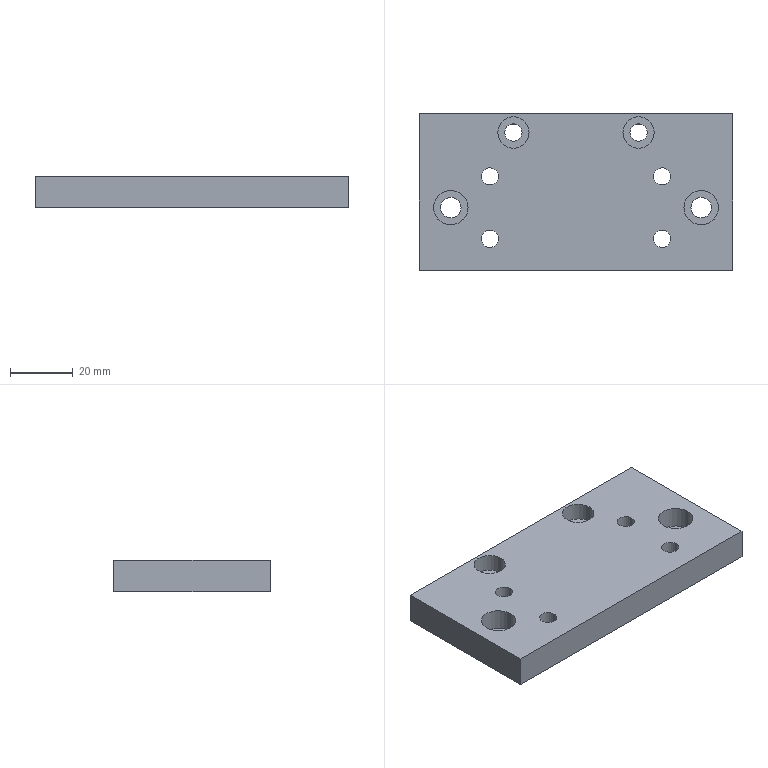Component | SolidWorks | 75-02-18StirringMotorMountingPlateModified-1 | 1 solid | 46 faces | box 100 x 50 x 10 mm | volume 45190 mm3 | cylinder 32 | plane 14 | commonest cylinder face diameters 10 x12 5.5 x12 11 x4 6.6 x4 | material A3 Steel
build123d program:
from build123d import *

# Parameters (mm, degrees)
SKETCH1_W                                          = 100
SKETCH1_H                                          = 50
BOSS_EXTRUDE1_DEPTH                                = 5
HOLE_SIZE_ACCORDING_TO_TYPE_OF_HEXAGON_D           = 5.5
HOLE_SIZE_ACCORDING_TO_TYPE_OF_HEXAGON_CBORE_D     = 10
HOLE_SIZE_ACCORDING_TO_TYPE_OF_HEXAGON_CBORE_DEPTH = 5.7
HOLE_SIZE_ACCORDING_TO_TYPE_OF_HEX_2_D             = 5.5
HOLE_SIZE_ACCORDING_TO_TYPE_OF_HEX_2_CBORE_D       = 10
HOLE_SIZE_ACCORDING_TO_TYPE_OF_HEX_2_CBORE_DEPTH   = 5.7
HOLE_SIZE_ACCORDING_TO_TYPE_OF_HEX_3_D             = 6.6
HOLE_SIZE_ACCORDING_TO_TYPE_OF_HEX_3_CBORE_D       = 11
HOLE_SIZE_ACCORDING_TO_TYPE_OF_HEX_3_CBORE_DEPTH   = 6.8


with BuildPart() as part:
    # Sketch1 → Boss-Extrude1 (new, symmetric)
    with BuildSketch(Plane.XY):
        Rectangle(SKETCH1_W, SKETCH1_H)
    extrude(amount=BOSS_EXTRUDE1_DEPTH, both=True)

    # Hole Size _according to_ Type of Hexagon (through all)
    with Locations(Plane(origin=(-27.5, 15, 5), x_dir=(1, 0, 0), z_dir=(0, 0, 1))):
        with Locations((0, 0), (0, -20), (55, 0), (55, -20)):
            CounterBoreHole(HOLE_SIZE_ACCORDING_TO_TYPE_OF_HEXAGON_D / 2, HOLE_SIZE_ACCORDING_TO_TYPE_OF_HEXAGON_CBORE_D / 2, HOLE_SIZE_ACCORDING_TO_TYPE_OF_HEXAGON_CBORE_DEPTH)

    # Hole Size _according to_ Type of Hex 2 (through all)
    with Locations(Plane(origin=(20, -19, -5), x_dir=(-1, 0, 0), z_dir=(0, 0, -1))):
        with Locations((0, 0), (40, 0)):
            CounterBoreHole(HOLE_SIZE_ACCORDING_TO_TYPE_OF_HEX_2_D / 2, HOLE_SIZE_ACCORDING_TO_TYPE_OF_HEX_2_CBORE_D / 2, HOLE_SIZE_ACCORDING_TO_TYPE_OF_HEX_2_CBORE_DEPTH)

    # Hole Size _according to_ Type of Hex 3 (through all)
    with Locations(Plane(origin=(40, 5, -5), x_dir=(-1, 0, 0), z_dir=(0, 0, -1))):
        with Locations((0, 0), (80, 0)):
            CounterBoreHole(HOLE_SIZE_ACCORDING_TO_TYPE_OF_HEX_3_D / 2, HOLE_SIZE_ACCORDING_TO_TYPE_OF_HEX_3_CBORE_D / 2, HOLE_SIZE_ACCORDING_TO_TYPE_OF_HEX_3_CBORE_DEPTH)


solid = part.part

# Placed as in the assembly
solid = solid.moved(Location((-17.8, 91.857, 7.75), (180, 0, 0)))